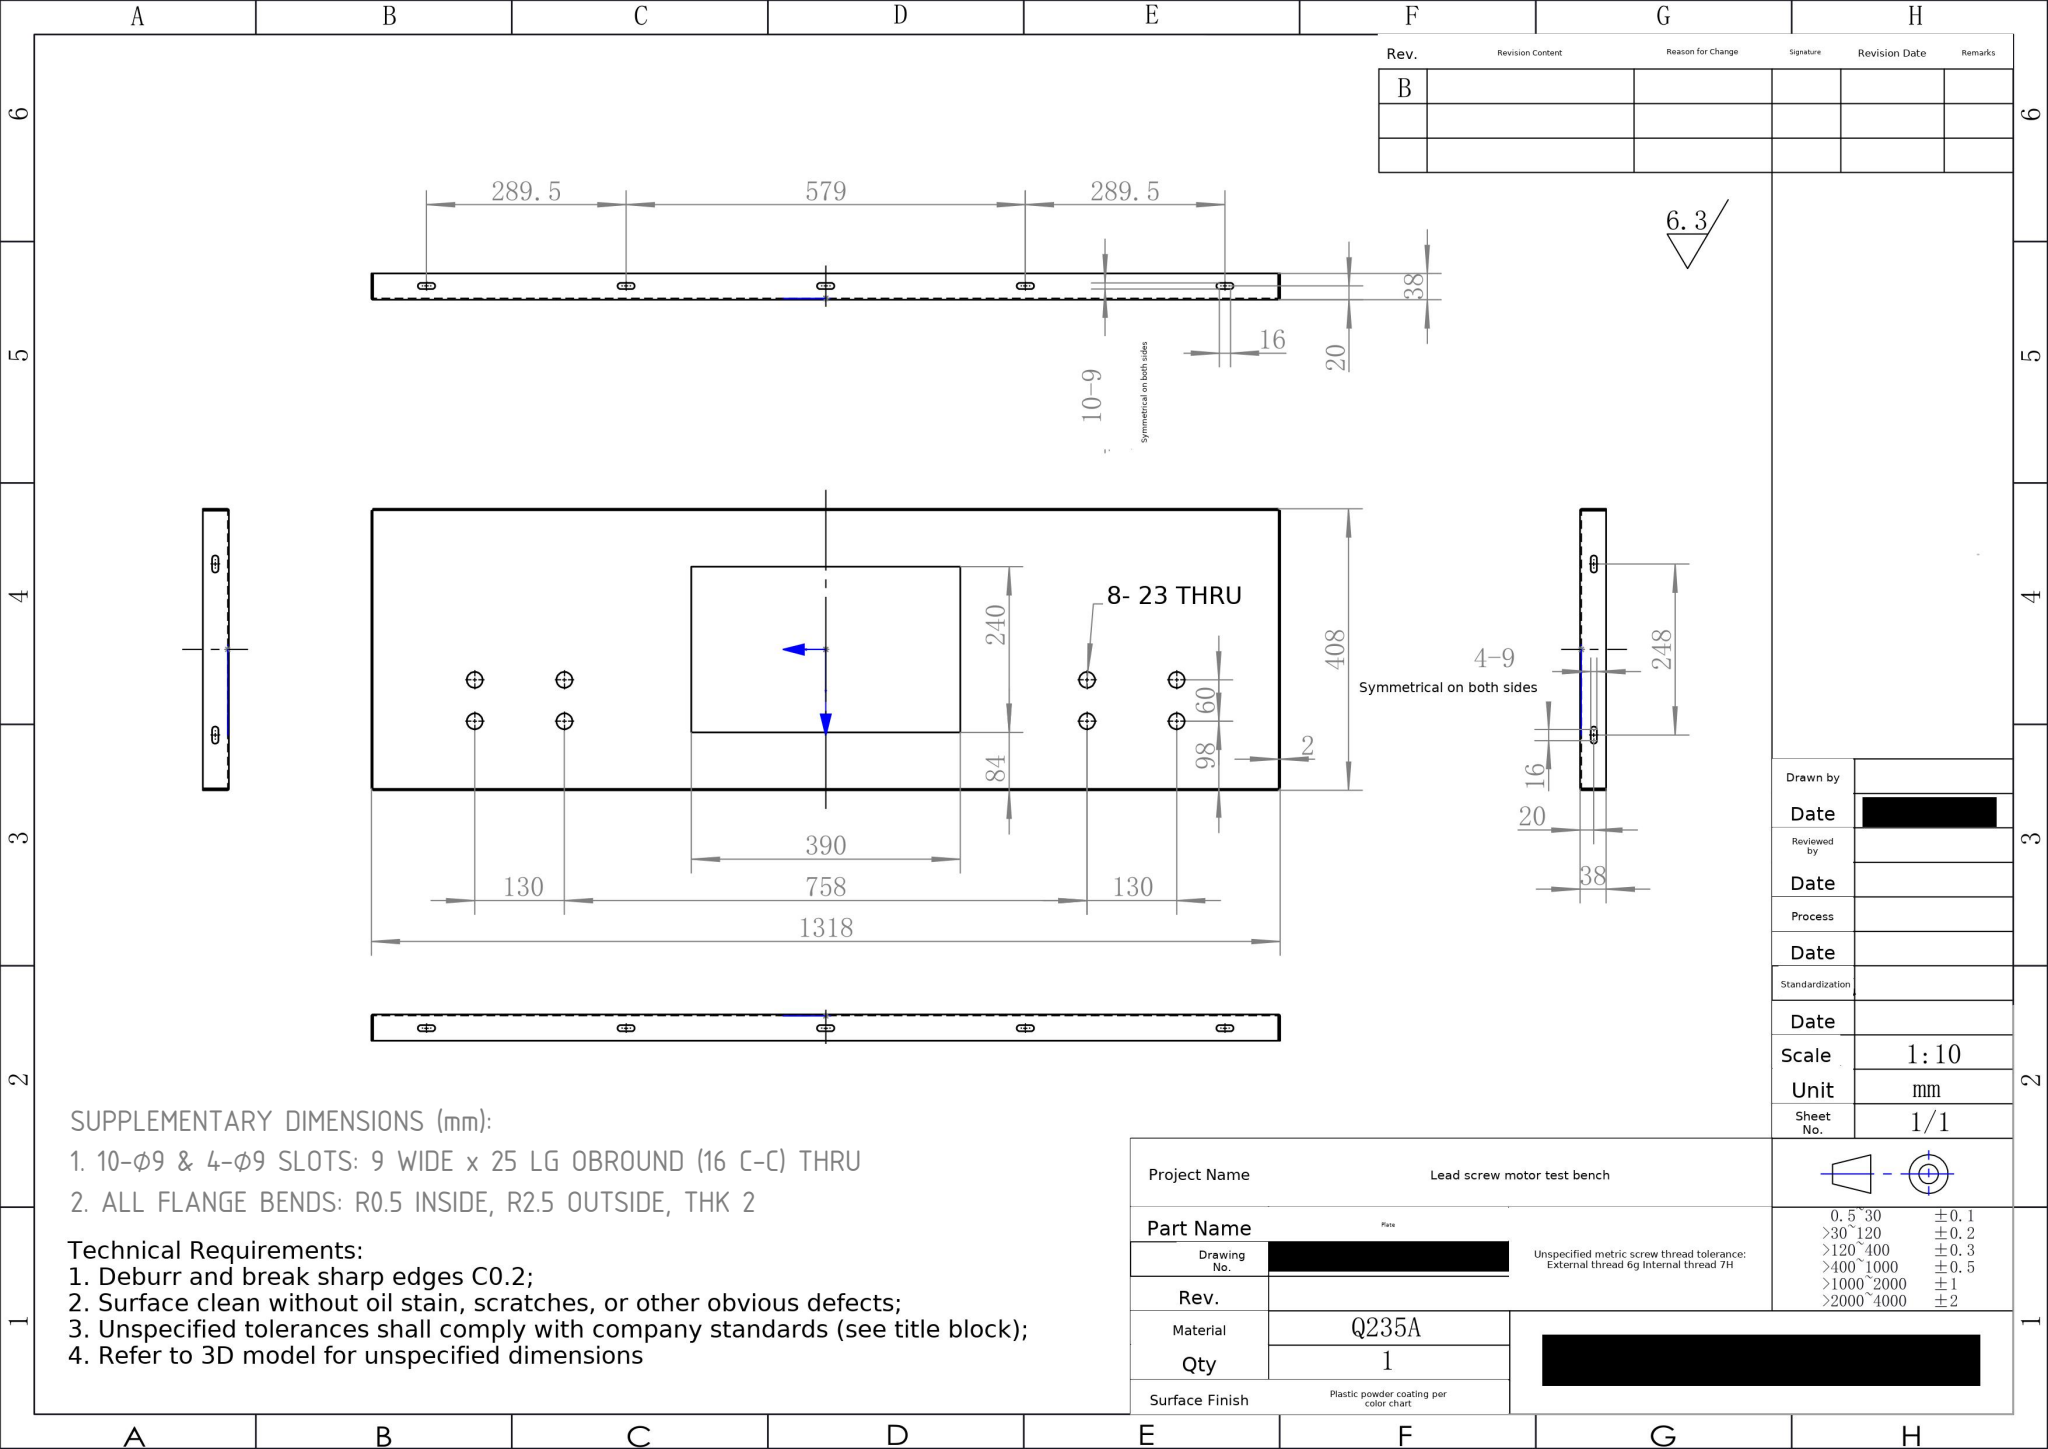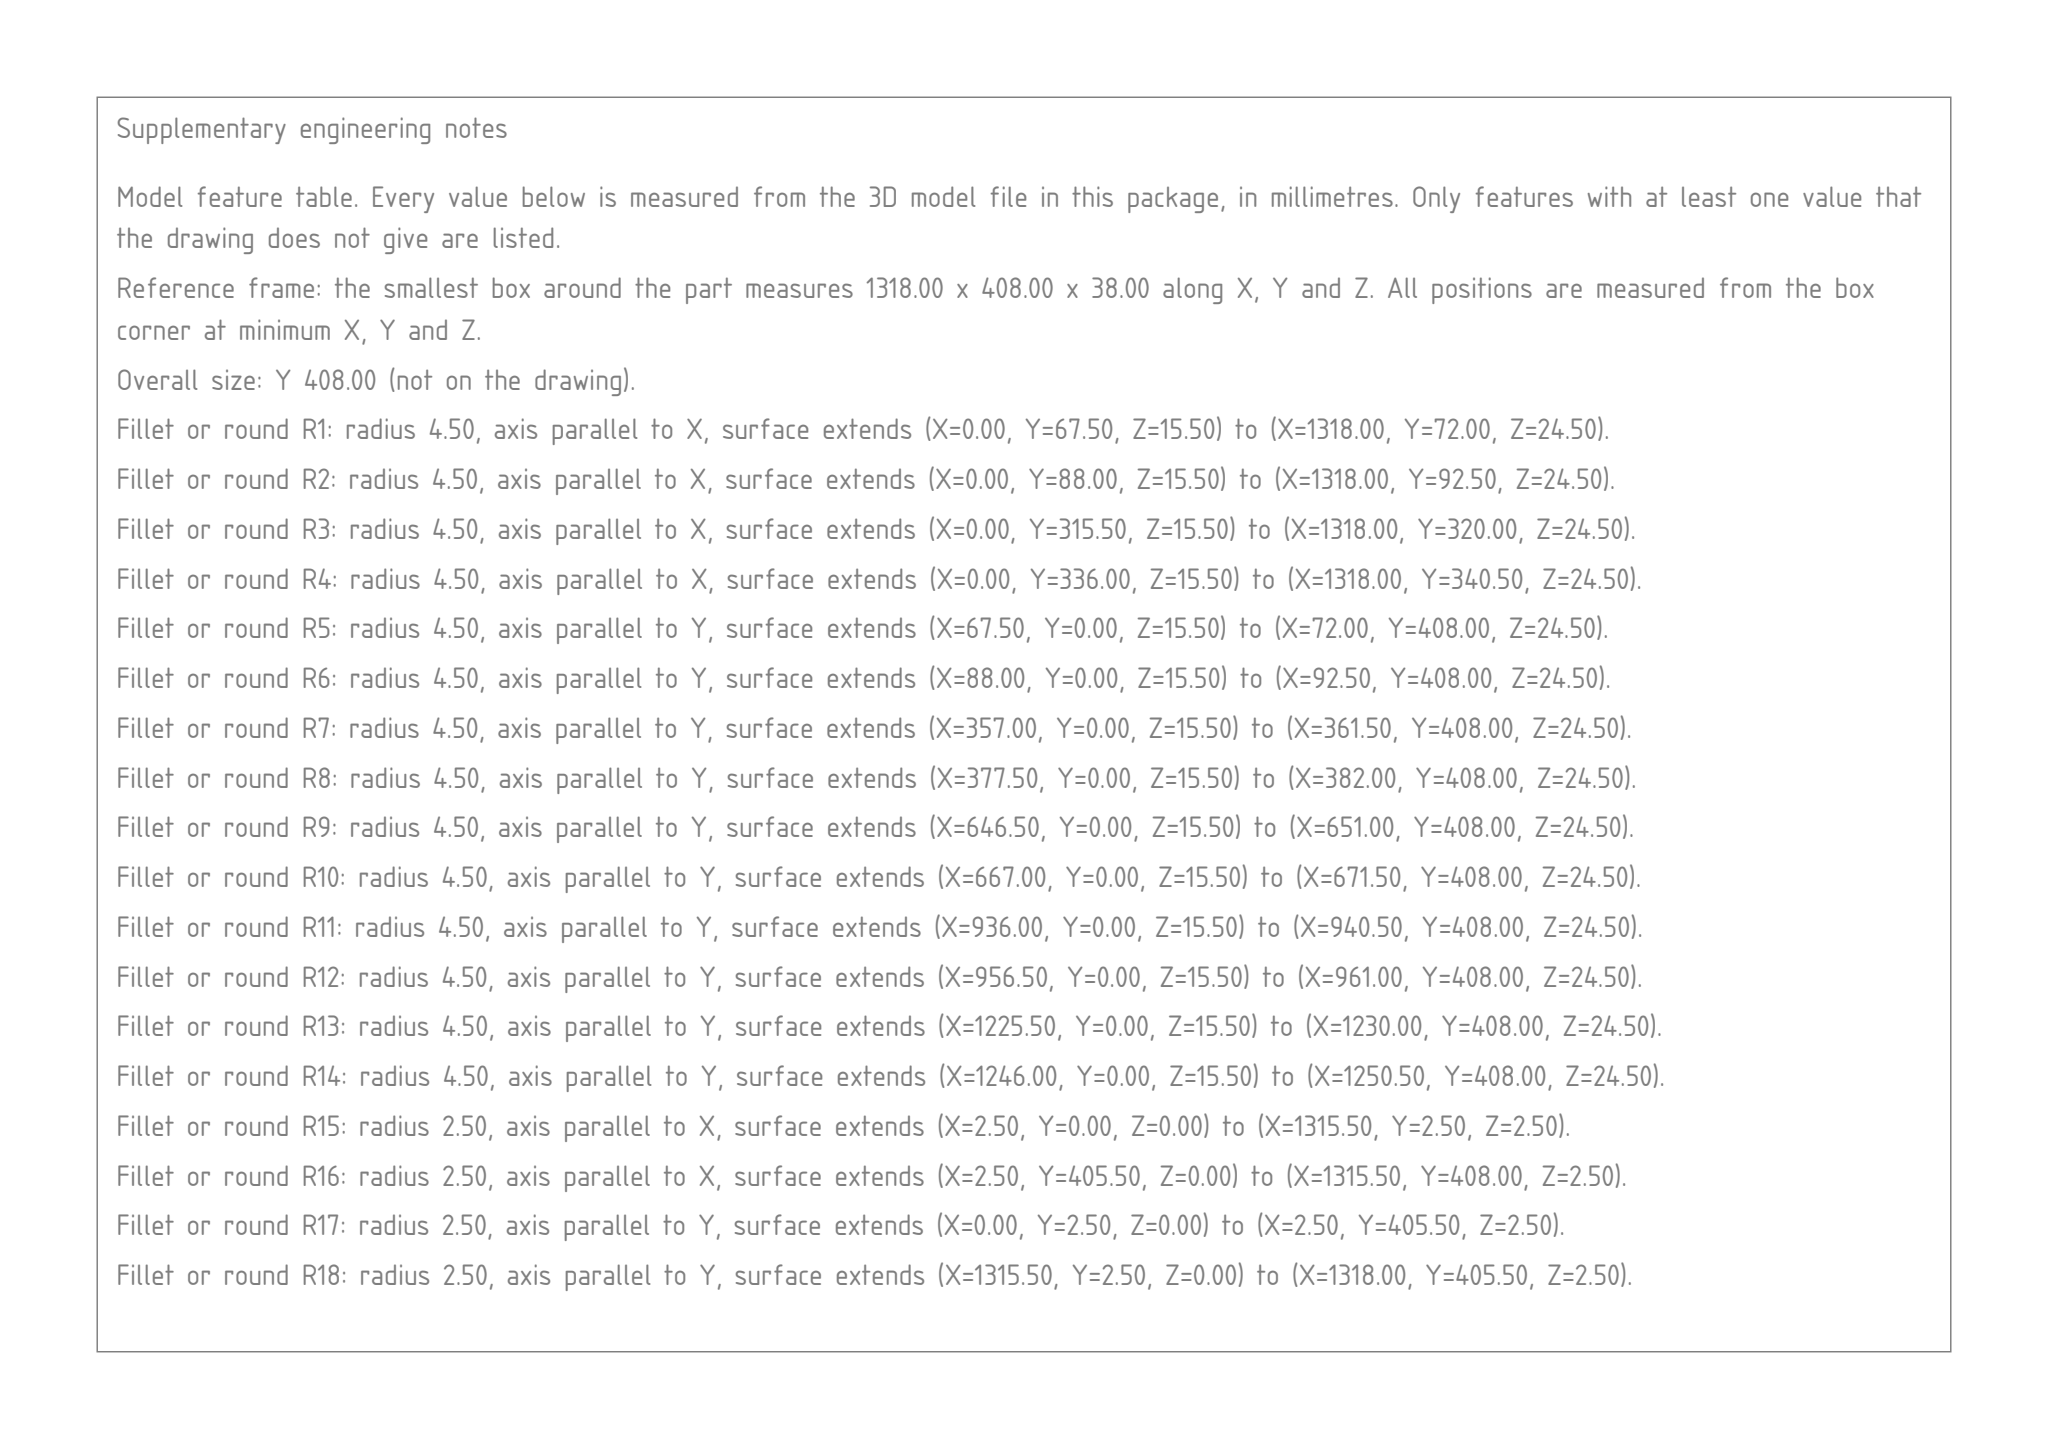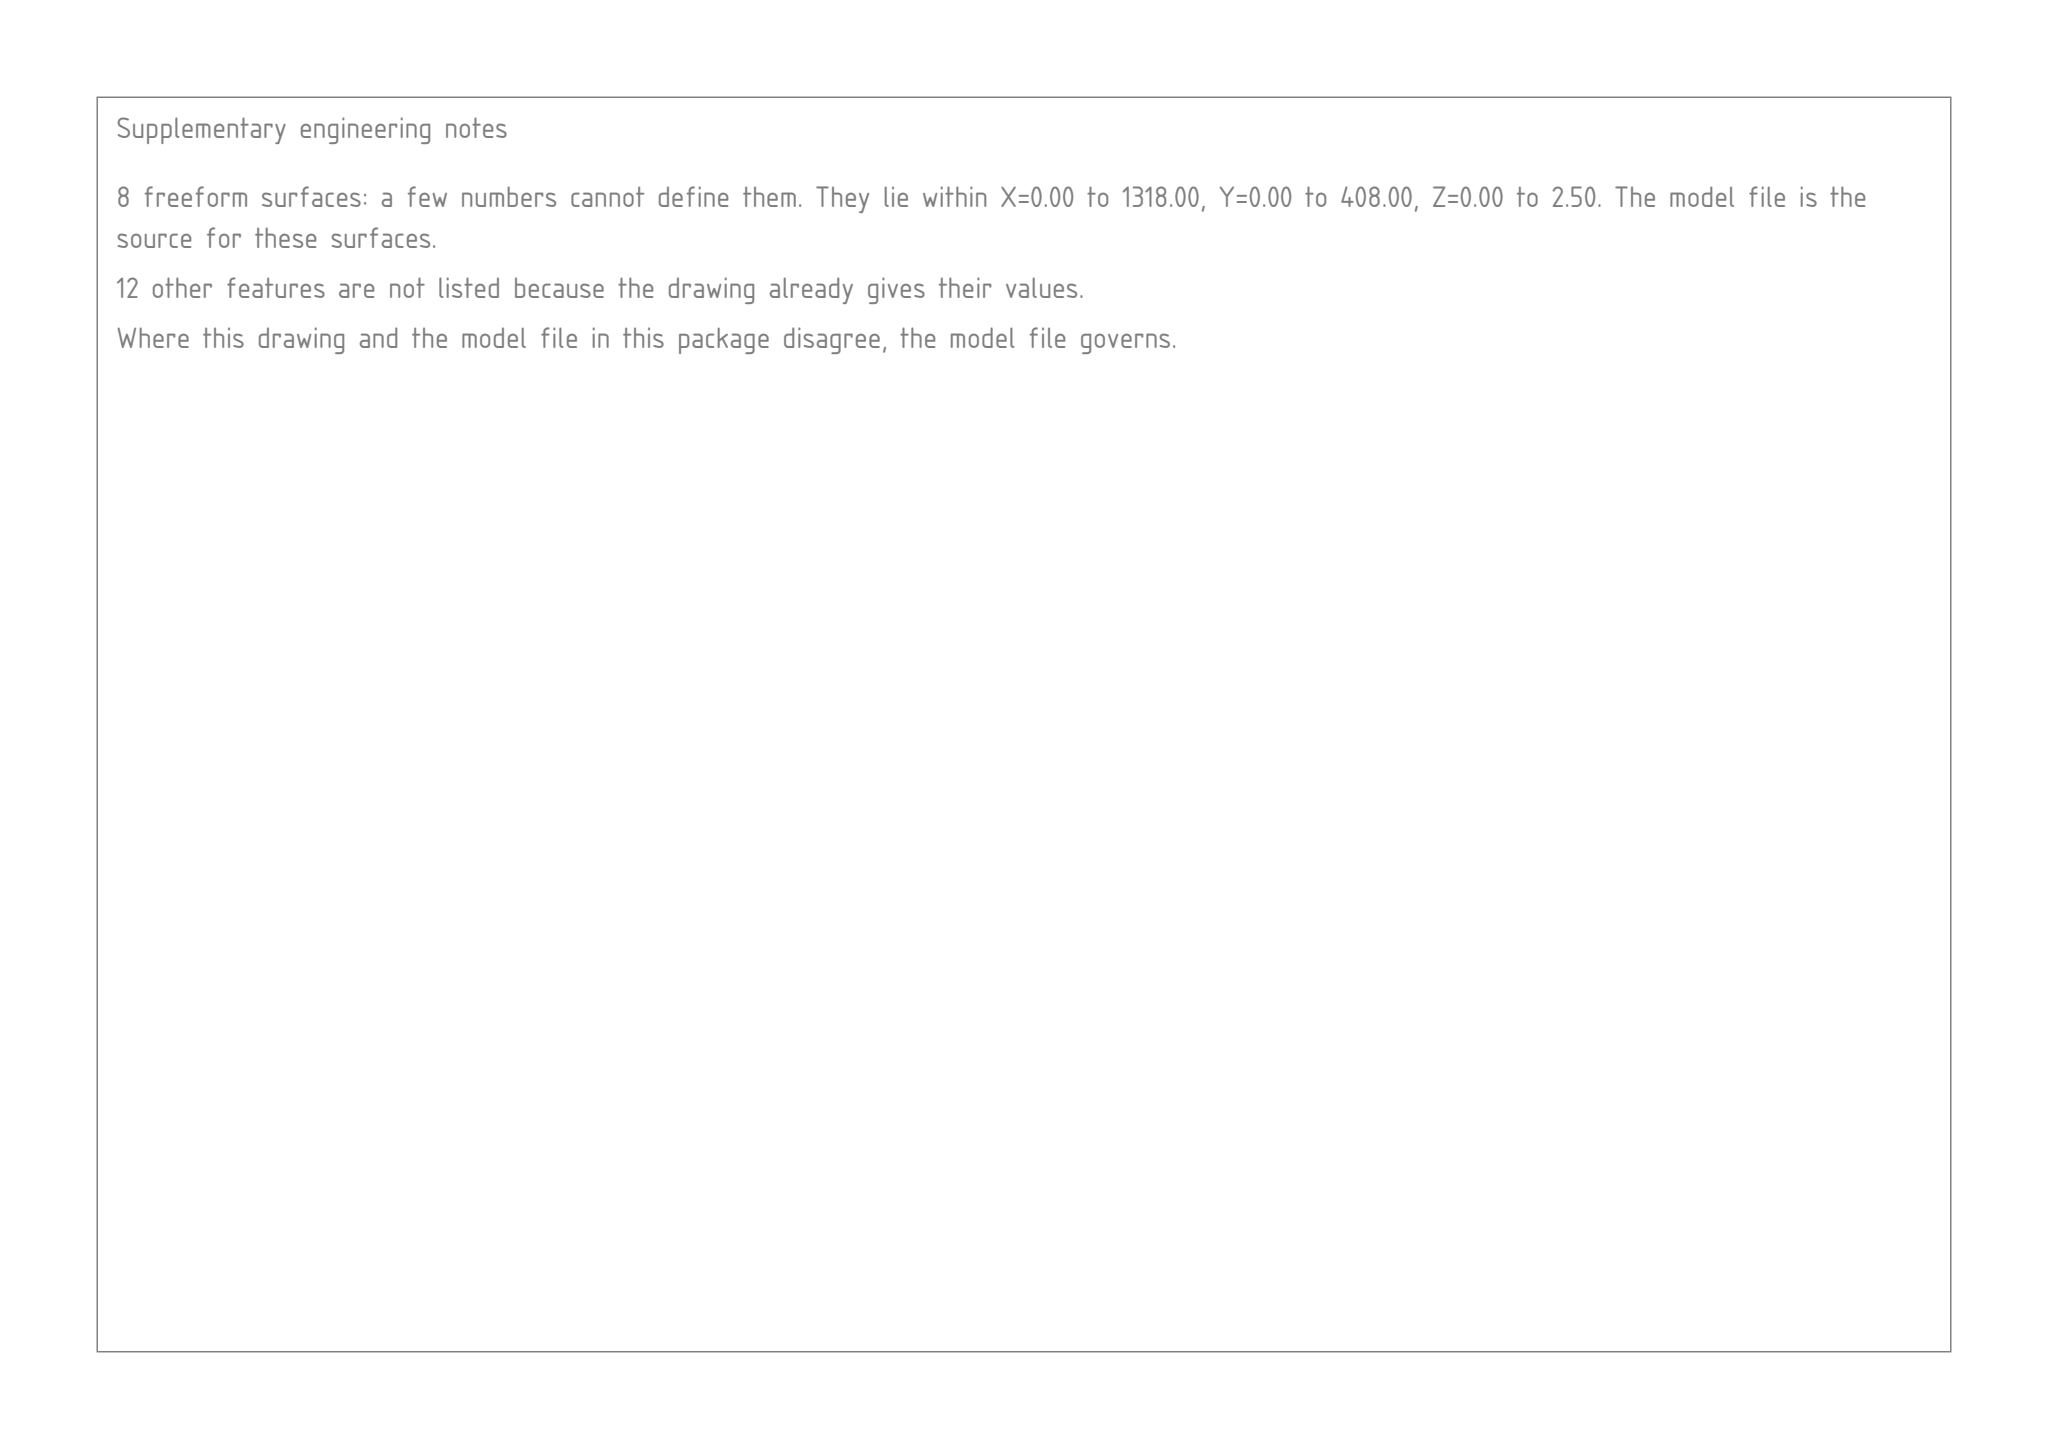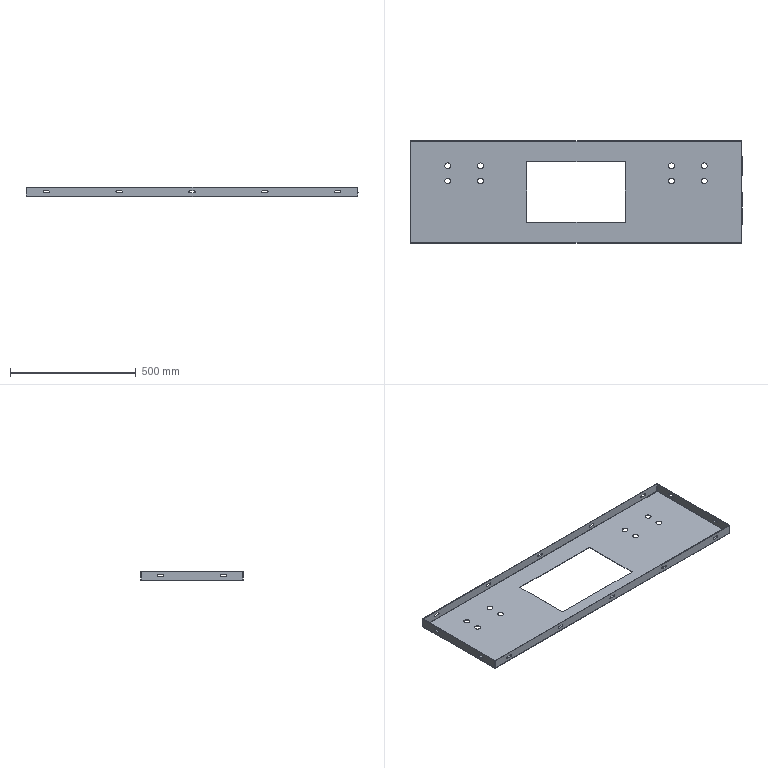Part | SolidWorks | mm | 1 solid | 114 faces | box 1318 x 408 x 38 mm | volume 1118340 mm3 | plane 54 | cylinder 52 | spline 8 | commonest cylinder face diameters 9 x28 23 x16 5 x4 1 x4